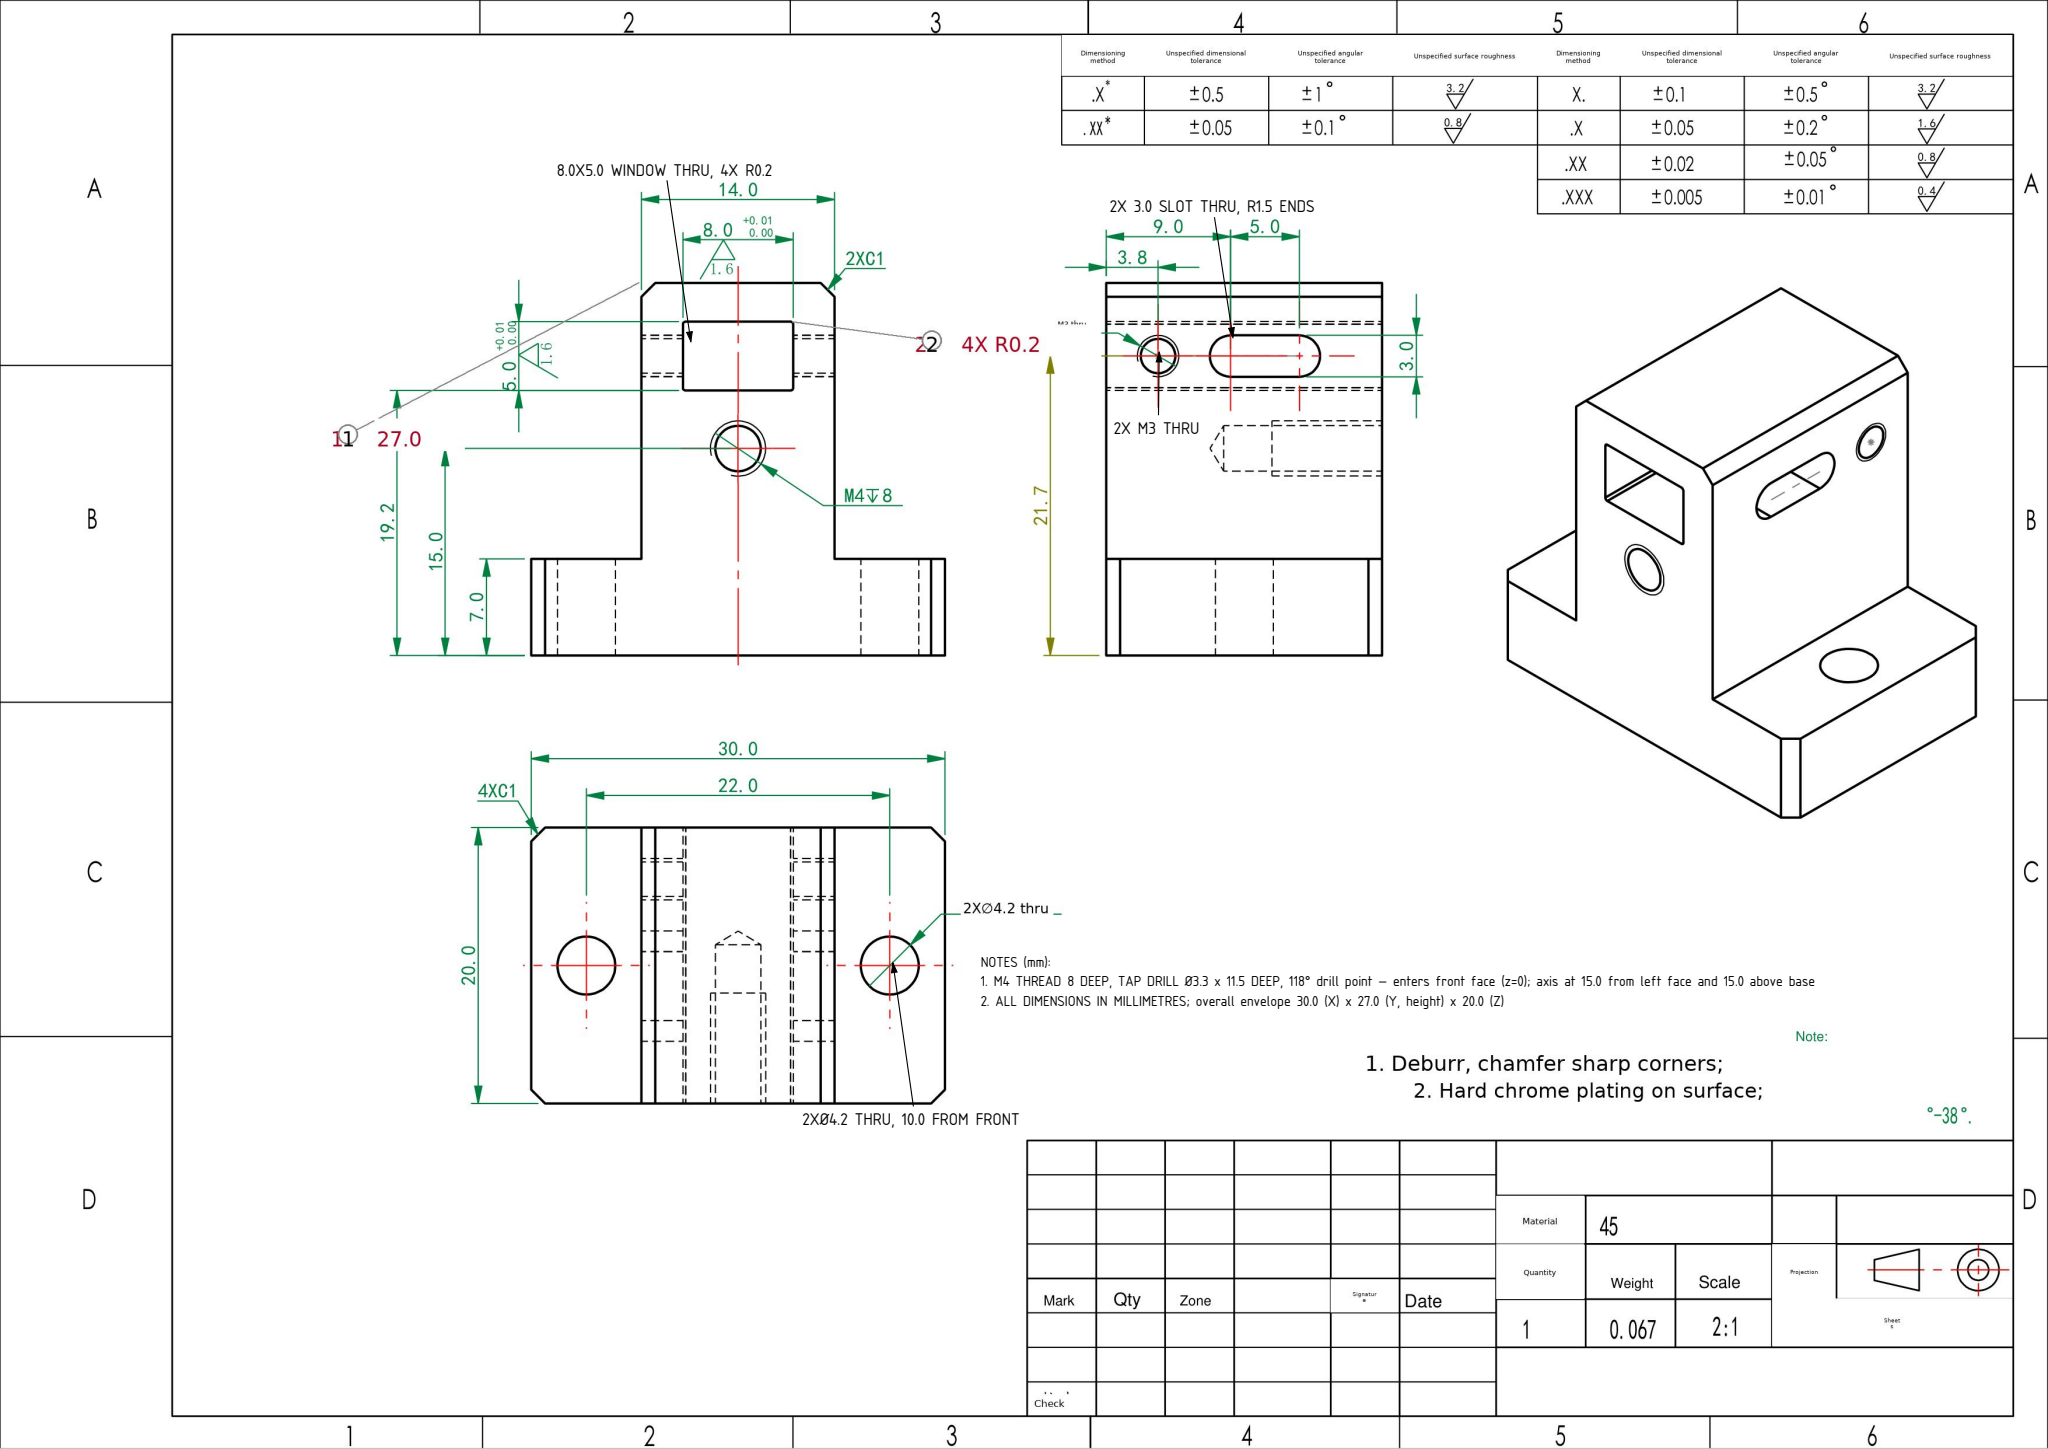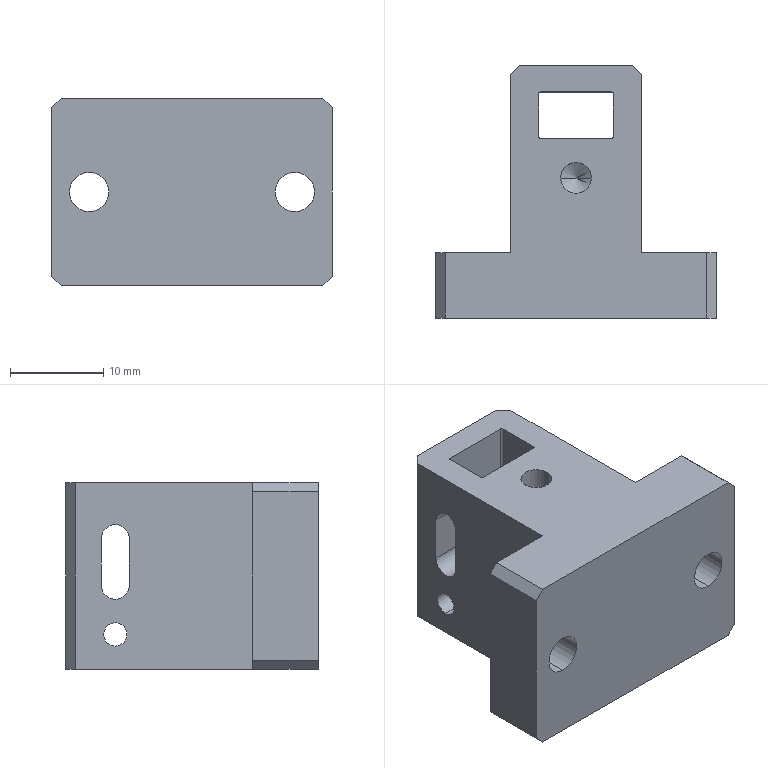Part | SolidWorks | mm | material 45 | 1 solid | 44 faces | box 30 x 27 x 20 mm | volume 8510 mm3 | plane 24 | cylinder 18 | cone 2 | commonest cylinder face diameters 2.5 x4 4.2 x4 3 x4 0.4 x4 3.3 x2
Drawing notes:
2X M3 THRU — one in each 3 mm thick side wall; axis 21.7 above base, 3.75 from front face (tap drill Ø2.5 x 3.0 thru wall) | from the solid: cylinders ⌀2.5 axis x at y=21.7, z=3.75, length 3.0 (side-wall thickness 3.0 from x-planes 8.0/11.0 and 19.0/22.0)
2X 3.0 WIDE OBROUND SLOT THRU — one in each 3 mm side wall; slot centerline 21.7 above base, end radii centers at 9.0 and 14.0 from front face (5.0 apart, R1.5 ends) | from the solid: cylinders ⌀3.0 axis x at y=21.7, z=9.0 and z=14.0, length 3.0, 2 each
8.0 x 5.0 RECTANGULAR WINDOW THRU upright wall; 11.0 to 19.0 from left face, 19.2 to 24.2 above base; 4X R0.2 corner reliefs | from the solid: x-planes 11.0/19.0, y-planes 19.2/24.2; ⌀0.4 z-cylinders at (11.2,19.4),(11.2,24.0),(18.8,19.4),(18.8,24.0) length 20.0
M4 THREAD 8 DEEP, TAP DRILL Ø3.3 x 11.5 DEEP, 118° drill point — enters front face (z=0); axis at 15.0 from left face and 15.0 above base | from the solid: cylinders ⌀3.3 axis z at x=15.0, y=15.0, length 11.5; cone 118° included angle, ref dia 3.3
2X Ø4.2 THRU base flange (7.0 thick); axes vertical through base at 4.0 and 26.0 from left face, 10.0 from front face | from the solid: cylinders ⌀4.2 axis y at (x=4.0, z=10.0) and (x=26.0, z=10.0), length 7.0; y-planes 0.0/7.0
ALL DIMENSIONS IN MILLIMETRES; overall envelope 30.0 (X) x 27.0 (Y, height) x 20.0 (Z) | from the solid: bbox_xyz [30.0, 27.0, 20.0], model units mm
build123d program:
from build123d import *

# Parameters (mm, degrees)
SKETCH1_W                  = 30
SKETCH1_H                  = 27
BOSS_EXTRUDE1_DEPTH        = 10
SKETCH2_W                  = 8
SKETCH2_H                  = 5
CUT_EXTRUDE1_DEPTH         = 23
CUT_EXTRUDE4_DEPTH         = 32
SKETCH7_W                  = 8
SKETCH7_H                  = 20
CUT_EXTRUDE6_DEPTH         = 20
F_4_2_4_2_DIAMETER_HOLE1_D = 4.2
M4_TAPPED_HOLE2_D          = 3.3
M4_TAPPED_HOLE2_DEPTH      = 11.5
M4_TAPPED_HOLE2_TIP        = 0.9914
CHAMFER1_SIZE              = 1
FILLET1_R                  = 0.2
CHAMFER2_SIZE              = 1
M3_TAPPED_HOLE1_D          = 2.5


with BuildPart() as part:
    # Sketch1 → Boss-Extrude1 (new, symmetric)
    with BuildSketch(Plane.XY):
        Rectangle(SKETCH1_W, SKETCH1_H)
    extrude(amount=BOSS_EXTRUDE1_DEPTH, both=True)

    # Sketch2 → Cut-Extrude1 (cut)
    with BuildSketch(Plane.XY.offset(10)):
        with Locations((0, 8.2)):
            Rectangle(SKETCH2_W, SKETCH2_H)
    extrude(amount=-CUT_EXTRUDE1_DEPTH, mode=Mode.SUBTRACT)

    # Sketch5 → Cut-Extrude4 (cut)
    with BuildSketch(Plane.ZY.offset(15)):
        with BuildLine():
            Line((-1, 9.7), (4, 9.7))
            ThreePointArc((4, 9.7), (5.5, 8.2), (4, 6.7))
            Line((4, 6.7), (-1, 6.7))
            ThreePointArc((-1, 6.7), (-2.5, 8.2), (-1, 9.7))
        make_face()
    extrude(amount=-CUT_EXTRUDE4_DEPTH, mode=Mode.SUBTRACT)

    # Sketch7 → Cut-Extrude6 (cut)
    with BuildSketch(Plane(origin=(0, 13.5, 0), x_dir=(1, 0, 0), z_dir=(0, 1, 0))):
        with Locations((-11, 0)):
            Rectangle(SKETCH7_W, SKETCH7_H)
        with Locations((11, 0)):
            Rectangle(SKETCH7_W, SKETCH7_H)
    extrude(amount=-CUT_EXTRUDE6_DEPTH, mode=Mode.SUBTRACT)

    # 4.2 _4.2_ Diameter Hole1 (through all)
    with Locations(Plane(origin=(-11, -6.5, 0), x_dir=(0, 0, 1), z_dir=(0, 1, 0))):
        with Locations((0, 0), (0, 22)):
            Hole(F_4_2_4_2_DIAMETER_HOLE1_D / 2)

    # M4 Tapped Hole2
    with Locations(Plane(origin=(0, 1.5, 10), x_dir=(1, 0, 0), z_dir=(0, 0, 1))):
        with Locations((0, 0)):
            Hole(M4_TAPPED_HOLE2_D / 2, depth=M4_TAPPED_HOLE2_DEPTH)
            with Locations((0, 0, -(M4_TAPPED_HOLE2_DEPTH + M4_TAPPED_HOLE2_TIP / 2))):  # 118° drill point
                Cone(0, M4_TAPPED_HOLE2_D / 2, M4_TAPPED_HOLE2_TIP, mode=Mode.SUBTRACT)

    # Chamfer1
    chamfer1_edges = [part.edges().sort_by_distance(p)[0] for p in [
        (15, -10, 10),
        (15, -10, -10),
        (-15, -10, -10),
        (-15, -10, 10),
    ]]
    chamfer(chamfer1_edges, length=CHAMFER1_SIZE)

    # Fillet1
    fillet1_edges = [part.edges().sort_by_distance(p)[0] for p in [
        (4, 10.7, 0),
        (4, 5.7, 0),
        (-4, 5.7, 0),
        (-4, 10.7, 0),
    ]]
    fillet(fillet1_edges, radius=FILLET1_R)

    # Chamfer2
    chamfer2_edges = [part.edges().sort_by_distance(p)[0] for p in [
        (-7, 13.5, 0),
        (7, 13.5, 0),
    ]]
    chamfer(chamfer2_edges, length=CHAMFER2_SIZE)

    # M3 Tapped Hole1 (through all)
    with Locations(Plane(origin=(7, 8.2, -6.25), x_dir=(0, 0, 1), z_dir=(1, 0, 0))):
        with Locations((0, 0)):
            Hole(M3_TAPPED_HOLE1_D / 2)


solid = part.part